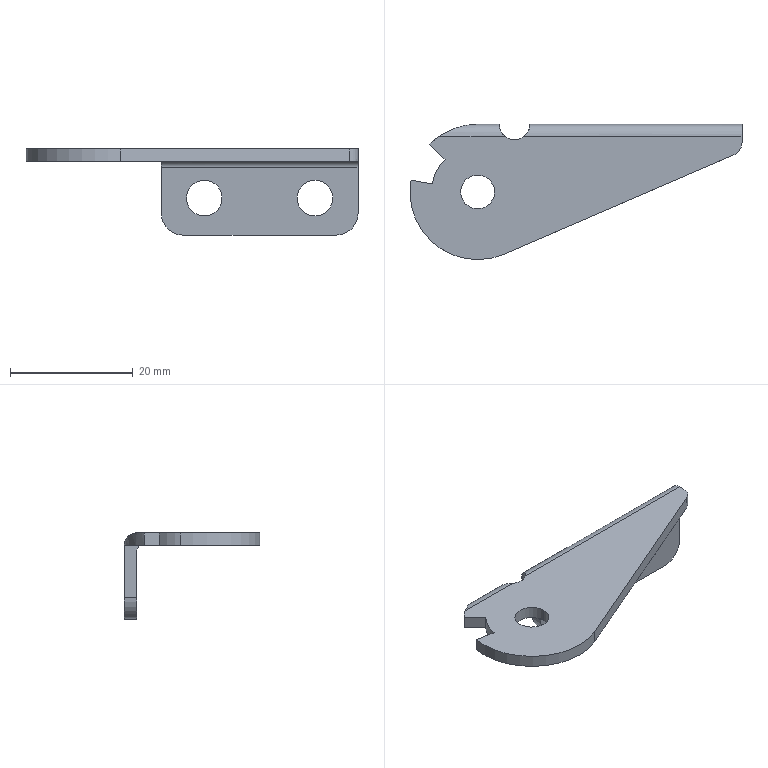Component | SolidWorks | MHPUS204-38-33-A-1_35-1 | 1 solid | 26 faces | box 54 x 22 x 14 mm | volume 2071 mm3 | cylinder 16 | plane 10 | commonest cylinder face diameters 5.8 x4 5.5 x2 4 x2 22 x2 7 x2 4.4 x1 15 x1 5 x1
STEP:
#1=COLOUR_RGB('',0.7922,0.8196,0.9333);
#2=FILL_AREA_STYLE_COLOUR('',#1);
#3=FILL_AREA_STYLE('',(#2));
#4=SURFACE_STYLE_FILL_AREA(#3);
#5=SURFACE_SIDE_STYLE('',(#4));
#6=SURFACE_STYLE_USAGE(.BOTH.,#5);
#7=PRESENTATION_STYLE_ASSIGNMENT((#6));
#8=CARTESIAN_POINT('',(20.594,-0.9055,3.138));
#9=VERTEX_POINT('',#8);
#10=CARTESIAN_POINT('',(20.81,-0.9055,3.138));
#11=VERTEX_POINT('',#10);
#12=CARTESIAN_POINT('',(20.702,-0.9055,3.138));
#13=DIRECTION('',(0.,0.,1.));
#14=DIRECTION('',(1.,0.,0.));
#15=AXIS2_PLACEMENT_3D('',#12,#13,#14);
#16=CIRCLE('',#15,0.1083);
#17=EDGE_CURVE('',#9,#11,#16,.T.);
#18=ORIENTED_EDGE('',*,*,#17,.F.);
#19=CARTESIAN_POINT('',(20.594,-0.9055,3.217));
#20=VERTEX_POINT('',#19);
#21=CARTESIAN_POINT('',(20.594,-0.9055,3.217));
#22=DIRECTION('',(0.,0.,1.));
#23=VECTOR('',#22,39.37);
#24=LINE('',#21,#23);
#25=EDGE_CURVE('',#9,#20,#24,.T.);
#26=ORIENTED_EDGE('',*,*,#25,.T.);
#27=CARTESIAN_POINT('',(20.81,-0.9055,3.217));
#28=VERTEX_POINT('',#27);
#29=CARTESIAN_POINT('',(20.702,-0.9055,3.217));
#30=DIRECTION('',(0.,0.,-1.));
#31=DIRECTION('',(1.,0.,0.));
#32=AXIS2_PLACEMENT_3D('',#29,#30,#31);
#33=CIRCLE('',#32,0.1083);
#34=EDGE_CURVE('',#28,#20,#33,.T.);
#35=ORIENTED_EDGE('',*,*,#34,.F.);
#36=CARTESIAN_POINT('',(20.81,-0.9055,3.217));
#37=DIRECTION('',(0.,0.,1.));
#38=VECTOR('',#37,39.37);
#39=LINE('',#36,#38);
#40=EDGE_CURVE('',#11,#28,#39,.T.);
#41=ORIENTED_EDGE('',*,*,#40,.F.);
#42=EDGE_LOOP('',(#18,#26,#35,#41));
#43=FACE_OUTER_BOUND('',#42,.T.);
#44=CARTESIAN_POINT('',(20.702,-0.9055,3.217));
#45=DIRECTION('',(0.,0.,1.));
#46=DIRECTION('',(1.,0.,0.));
#47=AXIS2_PLACEMENT_3D('',#44,#45,#46);
#48=CYLINDRICAL_SURFACE('',#47,0.1083);
#49=ADVANCED_FACE('',(#43),#48,.F.);
#50=CARTESIAN_POINT('',(21.411,-0.5512,2.787));
#51=VERTEX_POINT('',#50);
#52=CARTESIAN_POINT('',(21.411,-0.5512,3.016));
#53=VERTEX_POINT('',#52);
#54=CARTESIAN_POINT('',(21.411,-0.5512,2.902));
#55=DIRECTION('',(0.,1.,0.));
#56=DIRECTION('',(0.,0.,1.));
#57=AXIS2_PLACEMENT_3D('',#54,#55,#56);
#58=CIRCLE('',#57,0.1142);
#59=EDGE_CURVE('',#51,#53,#58,.T.);
#60=ORIENTED_EDGE('',*,*,#59,.F.);
#61=CARTESIAN_POINT('',(21.411,-0.4724,2.787));
#62=VERTEX_POINT('',#61);
#63=CARTESIAN_POINT('',(21.411,-0.3937,2.787));
#64=DIRECTION('',(0.,1.,0.));
#65=VECTOR('',#64,39.37);
#66=LINE('',#63,#65);
#67=EDGE_CURVE('',#51,#62,#66,.T.);
#68=ORIENTED_EDGE('',*,*,#67,.T.);
#69=CARTESIAN_POINT('',(21.411,-0.4724,3.016));
#70=VERTEX_POINT('',#69);
#71=CARTESIAN_POINT('',(21.411,-0.4724,2.902));
#72=DIRECTION('',(0.,-1.,0.));
#73=DIRECTION('',(0.,0.,1.));
#74=AXIS2_PLACEMENT_3D('',#71,#72,#73);
#75=CIRCLE('',#74,0.1142);
#76=EDGE_CURVE('',#70,#62,#75,.T.);
#77=ORIENTED_EDGE('',*,*,#76,.F.);
#78=CARTESIAN_POINT('',(21.411,-0.3937,3.016));
#79=DIRECTION('',(0.,1.,0.));
#80=VECTOR('',#79,39.37);
#81=LINE('',#78,#80);
#82=EDGE_CURVE('',#53,#70,#81,.T.);
#83=ORIENTED_EDGE('',*,*,#82,.F.);
#84=EDGE_LOOP('',(#60,#68,#77,#83));
#85=FACE_OUTER_BOUND('',#84,.T.);
#86=CARTESIAN_POINT('',(21.411,-0.3937,2.902));
#87=DIRECTION('',(0.,1.,0.));
#88=DIRECTION('',(0.,0.,1.));
#89=AXIS2_PLACEMENT_3D('',#86,#87,#88);
#90=CYLINDRICAL_SURFACE('',#89,0.1142);
#91=ADVANCED_FACE('',(#85),#90,.F.);
#92=CARTESIAN_POINT('',(22.119,-0.5512,2.787));
#93=VERTEX_POINT('',#92);
#94=CARTESIAN_POINT('',(22.119,-0.5512,3.016));
#95=VERTEX_POINT('',#94);
#96=CARTESIAN_POINT('',(22.119,-0.5512,2.902));
#97=DIRECTION('',(0.,1.,0.));
#98=DIRECTION('',(0.,0.,1.));
#99=AXIS2_PLACEMENT_3D('',#96,#97,#98);
#100=CIRCLE('',#99,0.1142);
#101=EDGE_CURVE('',#93,#95,#100,.T.);
#102=ORIENTED_EDGE('',*,*,#101,.F.);
#103=CARTESIAN_POINT('',(22.119,-0.4724,2.787));
#104=VERTEX_POINT('',#103);
#105=CARTESIAN_POINT('',(22.119,-0.3937,2.787));
#106=DIRECTION('',(0.,1.,0.));
#107=VECTOR('',#106,39.37);
#108=LINE('',#105,#107);
#109=EDGE_CURVE('',#93,#104,#108,.T.);
#110=ORIENTED_EDGE('',*,*,#109,.T.);
#111=CARTESIAN_POINT('',(22.119,-0.4724,3.016));
#112=VERTEX_POINT('',#111);
#113=CARTESIAN_POINT('',(22.119,-0.4724,2.902));
#114=DIRECTION('',(0.,-1.,0.));
#115=DIRECTION('',(0.,0.,1.));
#116=AXIS2_PLACEMENT_3D('',#113,#114,#115);
#117=CIRCLE('',#116,0.1142);
#118=EDGE_CURVE('',#112,#104,#117,.T.);
#119=ORIENTED_EDGE('',*,*,#118,.F.);
#120=CARTESIAN_POINT('',(22.119,-0.3937,3.016));
#121=DIRECTION('',(0.,1.,0.));
#122=VECTOR('',#121,39.37);
#123=LINE('',#120,#122);
#124=EDGE_CURVE('',#95,#112,#123,.T.);
#125=ORIENTED_EDGE('',*,*,#124,.F.);
#126=EDGE_LOOP('',(#102,#110,#119,#125));
#127=FACE_OUTER_BOUND('',#126,.T.);
#128=CARTESIAN_POINT('',(22.119,-0.3937,2.902));
#129=DIRECTION('',(0.,1.,0.));
#130=DIRECTION('',(0.,0.,1.));
#131=AXIS2_PLACEMENT_3D('',#128,#129,#130);
#132=CYLINDRICAL_SURFACE('',#131,0.1142);
#133=ADVANCED_FACE('',(#127),#132,.F.);
#134=CARTESIAN_POINT('',(22.395,-0.5512,3.217));
#135=VERTEX_POINT('',#134);
#136=CARTESIAN_POINT('',(22.395,-0.5887,3.217));
#137=VERTEX_POINT('',#136);
#138=CARTESIAN_POINT('',(22.395,-0.5887,3.217));
#139=DIRECTION('',(0.,-1.,0.));
#140=VECTOR('',#139,39.37);
#141=LINE('',#138,#140);
#142=EDGE_CURVE('',#135,#137,#141,.T.);
#143=ORIENTED_EDGE('',*,*,#142,.F.);
#144=CARTESIAN_POINT('',(20.997,-0.5512,3.217));
#145=VERTEX_POINT('',#144);
#146=CARTESIAN_POINT('',(20.702,-0.5512,3.217));
#147=DIRECTION('',(-1.,0.,0.));
#148=VECTOR('',#147,39.37);
#149=LINE('',#146,#148);
#150=EDGE_CURVE('',#135,#145,#149,.T.);
#151=ORIENTED_EDGE('',*,*,#150,.T.);
#152=CARTESIAN_POINT('',(20.879,-0.5512,3.217));
#153=VERTEX_POINT('',#152);
#154=CARTESIAN_POINT('',(20.938,-0.4724,3.217));
#155=DIRECTION('',(0.,0.,-1.));
#156=DIRECTION('',(1.,0.,0.));
#157=AXIS2_PLACEMENT_3D('',#154,#155,#156);
#158=CIRCLE('',#157,0.09843);
#159=EDGE_CURVE('',#145,#153,#158,.T.);
#160=ORIENTED_EDGE('',*,*,#159,.T.);
#161=CARTESIAN_POINT('',(20.453,-0.5512,3.217));
#162=VERTEX_POINT('',#161);
#163=CARTESIAN_POINT('',(20.702,-0.5512,3.217));
#164=DIRECTION('',(-1.,0.,0.));
#165=VECTOR('',#164,39.37);
#166=LINE('',#163,#165);
#167=EDGE_CURVE('',#153,#162,#166,.T.);
#168=ORIENTED_EDGE('',*,*,#167,.T.);
#169=CARTESIAN_POINT('',(20.396,-0.5993,3.217));
#170=VERTEX_POINT('',#169);
#171=CARTESIAN_POINT('',(20.702,-0.9055,3.217));
#172=DIRECTION('',(0.,0.,1.));
#173=DIRECTION('',(1.,0.,0.));
#174=AXIS2_PLACEMENT_3D('',#171,#172,#173);
#175=CIRCLE('',#174,0.4331);
#176=EDGE_CURVE('',#162,#170,#175,.T.);
#177=ORIENTED_EDGE('',*,*,#176,.T.);
#178=CARTESIAN_POINT('',(20.493,-0.6967,3.217));
#179=VERTEX_POINT('',#178);
#180=CARTESIAN_POINT('',(20.396,-0.5993,3.217));
#181=DIRECTION('',(0.7071,-0.7071,0.));
#182=VECTOR('',#181,39.37);
#183=LINE('',#180,#182);
#184=EDGE_CURVE('',#170,#179,#183,.T.);
#185=ORIENTED_EDGE('',*,*,#184,.T.);
#186=CARTESIAN_POINT('',(20.411,-0.8542,3.217));
#187=VERTEX_POINT('',#186);
#188=CARTESIAN_POINT('',(20.702,-0.9055,3.217));
#189=DIRECTION('',(0.,0.,1.));
#190=DIRECTION('',(1.,0.,0.));
#191=AXIS2_PLACEMENT_3D('',#188,#189,#190);
#192=CIRCLE('',#191,0.2953);
#193=EDGE_CURVE('',#179,#187,#192,.T.);
#194=ORIENTED_EDGE('',*,*,#193,.T.);
#195=CARTESIAN_POINT('',(20.276,-0.8303,3.217));
#196=VERTEX_POINT('',#195);
#197=CARTESIAN_POINT('',(20.411,-0.8542,3.217));
#198=DIRECTION('',(-0.9848,0.1736,0.));
#199=VECTOR('',#198,39.37);
#200=LINE('',#197,#199);
#201=EDGE_CURVE('',#187,#196,#200,.T.);
#202=ORIENTED_EDGE('',*,*,#201,.T.);
#203=CARTESIAN_POINT('',(20.874,-1.303,3.217));
#204=VERTEX_POINT('',#203);
#205=CARTESIAN_POINT('',(20.702,-0.9055,3.217));
#206=DIRECTION('',(0.,0.,1.));
#207=DIRECTION('',(1.,0.,0.));
#208=AXIS2_PLACEMENT_3D('',#205,#206,#207);
#209=CIRCLE('',#208,0.4331);
#210=EDGE_CURVE('',#196,#204,#209,.T.);
#211=ORIENTED_EDGE('',*,*,#210,.T.);
#212=CARTESIAN_POINT('',(22.343,-0.6683,3.217));
#213=VERTEX_POINT('',#212);
#214=CARTESIAN_POINT('',(20.874,-1.303,3.217));
#215=DIRECTION('',(0.9179,0.3967,0.));
#216=VECTOR('',#215,39.37);
#217=LINE('',#214,#216);
#218=EDGE_CURVE('',#204,#213,#217,.T.);
#219=ORIENTED_EDGE('',*,*,#218,.T.);
#220=CARTESIAN_POINT('',(22.308,-0.5887,3.217));
#221=DIRECTION('',(0.,0.,1.));
#222=DIRECTION('',(1.,0.,0.));
#223=AXIS2_PLACEMENT_3D('',#220,#221,#222);
#224=CIRCLE('',#223,0.08661);
#225=EDGE_CURVE('',#213,#137,#224,.T.);
#226=ORIENTED_EDGE('',*,*,#225,.T.);
#227=EDGE_LOOP('',(#143,#151,#160,#168,#177,#185,#194,#202,#211,#219,#226));
#228=FACE_OUTER_BOUND('',#227,.T.);
#229=ORIENTED_EDGE('',*,*,#34,.T.);
#230=CARTESIAN_POINT('',(20.702,-0.9055,3.217));
#231=DIRECTION('',(0.,0.,-1.));
#232=DIRECTION('',(1.,0.,0.));
#233=AXIS2_PLACEMENT_3D('',#230,#231,#232);
#234=CIRCLE('',#233,0.1083);
#235=EDGE_CURVE('',#20,#28,#234,.T.);
#236=ORIENTED_EDGE('',*,*,#235,.T.);
#237=EDGE_LOOP('',(#229,#236));
#238=FACE_BOUND('',#237,.T.);
#239=CARTESIAN_POINT('',(20.702,-1.339,3.217));
#240=DIRECTION('',(0.,0.,1.));
#241=DIRECTION('',(1.,0.,0.));
#242=AXIS2_PLACEMENT_3D('',#239,#240,#241);
#243=PLANE('',#242);
#244=ADVANCED_FACE('',(#228,#238),#243,.T.);
#245=CARTESIAN_POINT('',(22.395,-0.4724,3.138));
#246=VERTEX_POINT('',#245);
#247=CARTESIAN_POINT('',(21.135,-0.4724,3.138));
#248=VERTEX_POINT('',#247);
#249=CARTESIAN_POINT('',(23.261,-0.4724,3.138));
#250=DIRECTION('',(-1.,0.,0.));
#251=VECTOR('',#250,39.37);
#252=LINE('',#249,#251);
#253=EDGE_CURVE('',#246,#248,#252,.T.);
#254=ORIENTED_EDGE('',*,*,#253,.T.);
#255=CARTESIAN_POINT('',(21.037,-0.4724,3.138));
#256=VERTEX_POINT('',#255);
#257=CARTESIAN_POINT('',(23.261,-0.4724,3.138));
#258=DIRECTION('',(-1.,0.,0.));
#259=VECTOR('',#258,39.37);
#260=LINE('',#257,#259);
#261=EDGE_CURVE('',#248,#256,#260,.T.);
#262=ORIENTED_EDGE('',*,*,#261,.T.);
#263=CARTESIAN_POINT('',(21.037,-0.4724,3.138));
#264=CARTESIAN_POINT('',(21.037,-0.4724,3.143));
#265=CARTESIAN_POINT('',(21.037,-0.4731,3.149));
#266=CARTESIAN_POINT('',(21.037,-0.4755,3.16));
#267=CARTESIAN_POINT('',(21.037,-0.4773,3.166));
#268=CARTESIAN_POINT('',(21.036,-0.482,3.176));
#269=CARTESIAN_POINT('',(21.036,-0.4849,3.181));
#270=CARTESIAN_POINT('',(21.035,-0.4917,3.19));
#271=CARTESIAN_POINT('',(21.034,-0.4955,3.194));
#272=CARTESIAN_POINT('',(21.032,-0.5038,3.201));
#273=CARTESIAN_POINT('',(21.03,-0.5084,3.204));
#274=CARTESIAN_POINT('',(21.026,-0.5175,3.209));
#275=CARTESIAN_POINT('',(21.023,-0.5222,3.211));
#276=CARTESIAN_POINT('',(21.014,-0.5359,3.216));
#277=CARTESIAN_POINT('',(21.006,-0.5443,3.217));
#278=CARTESIAN_POINT('',(20.997,-0.5512,3.217));
#279=B_SPLINE_CURVE_WITH_KNOTS('',3,(#263,#264,#265,#266,#267,#268,#269,#270,#271,#272,#273,#274,#275,#276,#277,#278),.UNSPECIFIED.,.F.,.F.,(4,2,2,2,2,2,2,4),(0.,0.0004284,0.0008569,0.001285,0.001714,0.002142,0.002571,0.003428),.UNSPECIFIED.);
#280=EDGE_CURVE('',#256,#145,#279,.T.);
#281=ORIENTED_EDGE('',*,*,#280,.T.);
#282=ORIENTED_EDGE('',*,*,#150,.F.);
#283=CARTESIAN_POINT('',(22.395,-0.5512,3.138));
#284=DIRECTION('',(-1.,0.,0.));
#285=DIRECTION('',(0.,0.,-1.));
#286=AXIS2_PLACEMENT_3D('',#283,#284,#285);
#287=CIRCLE('',#286,0.07874);
#288=EDGE_CURVE('',#135,#246,#287,.T.);
#289=ORIENTED_EDGE('',*,*,#288,.T.);
#290=EDGE_LOOP('',(#254,#262,#281,#282,#289));
#291=FACE_OUTER_BOUND('',#290,.T.);
#292=CARTESIAN_POINT('',(23.261,-0.5512,3.138));
#293=DIRECTION('',(1.,0.,0.));
#294=DIRECTION('',(0.,0.,-1.));
#295=AXIS2_PLACEMENT_3D('',#292,#293,#294);
#296=CYLINDRICAL_SURFACE('',#295,0.07874);
#297=ADVANCED_FACE('',(#291),#296,.T.);
#298=CARTESIAN_POINT('',(22.343,-0.6683,3.138));
#299=VERTEX_POINT('',#298);
#300=CARTESIAN_POINT('',(22.343,-0.6683,3.217));
#301=DIRECTION('',(0.,0.,-1.));
#302=VECTOR('',#301,39.37);
#303=LINE('',#300,#302);
#304=EDGE_CURVE('',#213,#299,#303,.T.);
#305=ORIENTED_EDGE('',*,*,#304,.T.);
#306=CARTESIAN_POINT('',(22.395,-0.5906,3.138));
#307=VERTEX_POINT('',#306);
#308=CARTESIAN_POINT('',(22.308,-0.5887,3.138));
#309=DIRECTION('',(0.,0.,1.));
#310=DIRECTION('',(1.,0.,0.));
#311=AXIS2_PLACEMENT_3D('',#308,#309,#310);
#312=CIRCLE('',#311,0.08661);
#313=EDGE_CURVE('',#299,#307,#312,.T.);
#314=ORIENTED_EDGE('',*,*,#313,.T.);
#315=CARTESIAN_POINT('',(22.395,-0.5887,3.138));
#316=VERTEX_POINT('',#315);
#317=CARTESIAN_POINT('',(22.395,-0.5906,3.138));
#318=CARTESIAN_POINT('',(22.395,-0.5899,3.138));
#319=CARTESIAN_POINT('',(22.395,-0.5893,3.138));
#320=CARTESIAN_POINT('',(22.395,-0.5887,3.138));
#321=B_SPLINE_CURVE_WITH_KNOTS('',3,(#317,#318,#319,#320),.UNSPECIFIED.,.F.,.F.,(4,4),(0.,0.0000459),.UNSPECIFIED.);
#322=EDGE_CURVE('',#307,#316,#321,.T.);
#323=ORIENTED_EDGE('',*,*,#322,.T.);
#324=CARTESIAN_POINT('',(22.395,-0.5887,3.217));
#325=DIRECTION('',(0.,0.,1.));
#326=VECTOR('',#325,39.37);
#327=LINE('',#324,#326);
#328=EDGE_CURVE('',#316,#137,#327,.T.);
#329=ORIENTED_EDGE('',*,*,#328,.T.);
#330=ORIENTED_EDGE('',*,*,#225,.F.);
#331=EDGE_LOOP('',(#305,#314,#323,#329,#330));
#332=FACE_OUTER_BOUND('',#331,.T.);
#333=CARTESIAN_POINT('',(22.308,-0.5887,3.217));
#334=DIRECTION('',(0.,0.,1.));
#335=DIRECTION('',(1.,0.,0.));
#336=AXIS2_PLACEMENT_3D('',#333,#334,#335);
#337=CYLINDRICAL_SURFACE('',#336,0.08661);
#338=ADVANCED_FACE('',(#332),#337,.T.);
#339=ORIENTED_EDGE('',*,*,#218,.F.);
#340=CARTESIAN_POINT('',(20.874,-1.303,3.138));
#341=VERTEX_POINT('',#340);
#342=CARTESIAN_POINT('',(20.874,-1.303,3.217));
#343=DIRECTION('',(0.,0.,-1.));
#344=VECTOR('',#343,39.37);
#345=LINE('',#342,#344);
#346=EDGE_CURVE('',#204,#341,#345,.T.);
#347=ORIENTED_EDGE('',*,*,#346,.T.);
#348=CARTESIAN_POINT('',(20.874,-1.303,3.138));
#349=DIRECTION('',(0.9179,0.3967,0.));
#350=VECTOR('',#349,39.37);
#351=LINE('',#348,#350);
#352=EDGE_CURVE('',#341,#299,#351,.T.);
#353=ORIENTED_EDGE('',*,*,#352,.T.);
#354=ORIENTED_EDGE('',*,*,#304,.F.);
#355=EDGE_LOOP('',(#339,#347,#353,#354));
#356=FACE_OUTER_BOUND('',#355,.T.);
#357=CARTESIAN_POINT('',(20.874,-1.303,3.217));
#358=DIRECTION('',(0.3967,-0.9179,0.));
#359=DIRECTION('',(0.9179,0.3967,0.));
#360=AXIS2_PLACEMENT_3D('',#357,#358,#359);
#361=PLANE('',#360);
#362=ADVANCED_FACE('',(#356),#361,.T.);
#363=ORIENTED_EDGE('',*,*,#210,.F.);
#364=CARTESIAN_POINT('',(20.276,-0.8303,3.138));
#365=VERTEX_POINT('',#364);
#366=CARTESIAN_POINT('',(20.276,-0.8303,3.217));
#367=DIRECTION('',(0.,0.,-1.));
#368=VECTOR('',#367,39.37);
#369=LINE('',#366,#368);
#370=EDGE_CURVE('',#196,#365,#369,.T.);
#371=ORIENTED_EDGE('',*,*,#370,.T.);
#372=CARTESIAN_POINT('',(20.702,-0.9055,3.138));
#373=DIRECTION('',(0.,0.,1.));
#374=DIRECTION('',(1.,0.,0.));
#375=AXIS2_PLACEMENT_3D('',#372,#373,#374);
#376=CIRCLE('',#375,0.4331);
#377=EDGE_CURVE('',#365,#341,#376,.T.);
#378=ORIENTED_EDGE('',*,*,#377,.T.);
#379=ORIENTED_EDGE('',*,*,#346,.F.);
#380=EDGE_LOOP('',(#363,#371,#378,#379));
#381=FACE_OUTER_BOUND('',#380,.T.);
#382=CARTESIAN_POINT('',(20.702,-0.9055,3.217));
#383=DIRECTION('',(0.,0.,1.));
#384=DIRECTION('',(1.,0.,0.));
#385=AXIS2_PLACEMENT_3D('',#382,#383,#384);
#386=CYLINDRICAL_SURFACE('',#385,0.4331);
#387=ADVANCED_FACE('',(#381),#386,.T.);
#388=ORIENTED_EDGE('',*,*,#201,.F.);
#389=CARTESIAN_POINT('',(20.411,-0.8542,3.138));
#390=VERTEX_POINT('',#389);
#391=CARTESIAN_POINT('',(20.411,-0.8542,3.217));
#392=DIRECTION('',(0.,0.,-1.));
#393=VECTOR('',#392,39.37);
#394=LINE('',#391,#393);
#395=EDGE_CURVE('',#187,#390,#394,.T.);
#396=ORIENTED_EDGE('',*,*,#395,.T.);
#397=CARTESIAN_POINT('',(20.411,-0.8542,3.138));
#398=DIRECTION('',(-0.9848,0.1736,0.));
#399=VECTOR('',#398,39.37);
#400=LINE('',#397,#399);
#401=EDGE_CURVE('',#390,#365,#400,.T.);
#402=ORIENTED_EDGE('',*,*,#401,.T.);
#403=ORIENTED_EDGE('',*,*,#370,.F.);
#404=EDGE_LOOP('',(#388,#396,#402,#403));
#405=FACE_OUTER_BOUND('',#404,.T.);
#406=CARTESIAN_POINT('',(20.411,-0.8542,3.217));
#407=DIRECTION('',(0.1736,0.9848,0.));
#408=DIRECTION('',(-0.9848,0.1736,0.));
#409=AXIS2_PLACEMENT_3D('',#406,#407,#408);
#410=PLANE('',#409);
#411=ADVANCED_FACE('',(#405),#410,.T.);
#412=ORIENTED_EDGE('',*,*,#193,.F.);
#413=CARTESIAN_POINT('',(20.493,-0.6967,3.138));
#414=VERTEX_POINT('',#413);
#415=CARTESIAN_POINT('',(20.493,-0.6967,3.217));
#416=DIRECTION('',(0.,0.,-1.));
#417=VECTOR('',#416,39.37);
#418=LINE('',#415,#417);
#419=EDGE_CURVE('',#179,#414,#418,.T.);
#420=ORIENTED_EDGE('',*,*,#419,.T.);
#421=CARTESIAN_POINT('',(20.702,-0.9055,3.138));
#422=DIRECTION('',(0.,0.,1.));
#423=DIRECTION('',(1.,0.,0.));
#424=AXIS2_PLACEMENT_3D('',#421,#422,#423);
#425=CIRCLE('',#424,0.2953);
#426=EDGE_CURVE('',#414,#390,#425,.T.);
#427=ORIENTED_EDGE('',*,*,#426,.T.);
#428=ORIENTED_EDGE('',*,*,#395,.F.);
#429=EDGE_LOOP('',(#412,#420,#427,#428));
#430=FACE_OUTER_BOUND('',#429,.T.);
#431=CARTESIAN_POINT('',(20.702,-0.9055,3.217));
#432=DIRECTION('',(0.,0.,1.));
#433=DIRECTION('',(1.,0.,0.));
#434=AXIS2_PLACEMENT_3D('',#431,#432,#433);
#435=CYLINDRICAL_SURFACE('',#434,0.2953);
#436=ADVANCED_FACE('',(#430),#435,.T.);
#437=ORIENTED_EDGE('',*,*,#184,.F.);
#438=CARTESIAN_POINT('',(20.396,-0.5993,3.138));
#439=VERTEX_POINT('',#438);
#440=CARTESIAN_POINT('',(20.396,-0.5993,3.217));
#441=DIRECTION('',(0.,0.,-1.));
#442=VECTOR('',#441,39.37);
#443=LINE('',#440,#442);
#444=EDGE_CURVE('',#170,#439,#443,.T.);
#445=ORIENTED_EDGE('',*,*,#444,.T.);
#446=CARTESIAN_POINT('',(20.396,-0.5993,3.138));
#447=DIRECTION('',(0.7071,-0.7071,0.));
#448=VECTOR('',#447,39.37);
#449=LINE('',#446,#448);
#450=EDGE_CURVE('',#439,#414,#449,.T.);
#451=ORIENTED_EDGE('',*,*,#450,.T.);
#452=ORIENTED_EDGE('',*,*,#419,.F.);
#453=EDGE_LOOP('',(#437,#445,#451,#452));
#454=FACE_OUTER_BOUND('',#453,.T.);
#455=CARTESIAN_POINT('',(20.396,-0.5993,3.217));
#456=DIRECTION('',(-0.7071,-0.7071,0.));
#457=DIRECTION('',(0.7071,-0.7071,0.));
#458=AXIS2_PLACEMENT_3D('',#455,#456,#457);
#459=PLANE('',#458);
#460=ADVANCED_FACE('',(#454),#459,.T.);
#461=ORIENTED_EDGE('',*,*,#176,.F.);
#462=CARTESIAN_POINT('',(20.702,-0.4724,3.138));
#463=VERTEX_POINT('',#462);
#464=CARTESIAN_POINT('',(20.453,-0.5512,3.217));
#465=CARTESIAN_POINT('',(20.472,-0.5377,3.217));
#466=CARTESIAN_POINT('',(20.492,-0.5261,3.213));
#467=CARTESIAN_POINT('',(20.523,-0.5111,3.206));
#468=CARTESIAN_POINT('',(20.533,-0.5066,3.203));
#469=CARTESIAN_POINT('',(20.554,-0.4984,3.196));
#470=CARTESIAN_POINT('',(20.564,-0.4948,3.193));
#471=CARTESIAN_POINT('',(20.596,-0.4852,3.182));
#472=CARTESIAN_POINT('',(20.617,-0.4804,3.174));
#473=CARTESIAN_POINT('',(20.649,-0.4756,3.16));
#474=CARTESIAN_POINT('',(20.659,-0.4744,3.156));
#475=CARTESIAN_POINT('',(20.681,-0.4728,3.147));
#476=CARTESIAN_POINT('',(20.691,-0.4724,3.142));
#477=CARTESIAN_POINT('',(20.702,-0.4724,3.138));
#478=B_SPLINE_CURVE_WITH_KNOTS('',3,(#464,#465,#466,#467,#468,#469,#470,#471,#472,#473,#474,#475,#476,#477),.UNSPECIFIED.,.F.,.F.,(4,2,2,2,2,2,4),(0.,0.001765,0.002648,0.003531,0.005296,0.006179,0.007061),.UNSPECIFIED.);
#479=EDGE_CURVE('',#162,#463,#478,.T.);
#480=ORIENTED_EDGE('',*,*,#479,.T.);
#481=CARTESIAN_POINT('',(20.702,-0.9055,3.138));
#482=DIRECTION('',(0.,0.,1.));
#483=DIRECTION('',(1.,0.,0.));
#484=AXIS2_PLACEMENT_3D('',#481,#482,#483);
#485=CIRCLE('',#484,0.4331);
#486=EDGE_CURVE('',#463,#439,#485,.T.);
#487=ORIENTED_EDGE('',*,*,#486,.T.);
#488=ORIENTED_EDGE('',*,*,#444,.F.);
#489=EDGE_LOOP('',(#461,#480,#487,#488));
#490=FACE_OUTER_BOUND('',#489,.T.);
#491=CARTESIAN_POINT('',(20.702,-0.9055,3.217));
#492=DIRECTION('',(0.,0.,1.));
#493=DIRECTION('',(1.,0.,0.));
#494=AXIS2_PLACEMENT_3D('',#491,#492,#493);
#495=CYLINDRICAL_SURFACE('',#494,0.4331);
#496=ADVANCED_FACE('',(#490),#495,.T.);
#497=ORIENTED_EDGE('',*,*,#479,.F.);
#498=ORIENTED_EDGE('',*,*,#167,.F.);
#499=CARTESIAN_POINT('',(20.84,-0.4724,3.138));
#500=VERTEX_POINT('',#499);
#501=CARTESIAN_POINT('',(20.879,-0.5512,3.217));
#502=CARTESIAN_POINT('',(20.875,-0.5478,3.217));
#503=CARTESIAN_POINT('',(20.871,-0.544,3.216));
#504=CARTESIAN_POINT('',(20.863,-0.5359,3.215));
#505=CARTESIAN_POINT('',(20.859,-0.5314,3.214));
#506=CARTESIAN_POINT('',(20.853,-0.5224,3.211));
#507=CARTESIAN_POINT('',(20.851,-0.5177,3.209));
#508=CARTESIAN_POINT('',(20.847,-0.5085,3.204));
#509=CARTESIAN_POINT('',(20.845,-0.504,3.201));
#510=CARTESIAN_POINT('',(20.843,-0.4957,3.194));
#511=CARTESIAN_POINT('',(20.842,-0.4917,3.19));
#512=CARTESIAN_POINT('',(20.841,-0.485,3.181));
#513=CARTESIAN_POINT('',(20.84,-0.482,3.176));
#514=CARTESIAN_POINT('',(20.84,-0.4773,3.166));
#515=CARTESIAN_POINT('',(20.84,-0.4755,3.16));
#516=CARTESIAN_POINT('',(20.84,-0.4731,3.149));
#517=CARTESIAN_POINT('',(20.84,-0.4724,3.143));
#518=CARTESIAN_POINT('',(20.84,-0.4724,3.138));
#519=B_SPLINE_CURVE_WITH_KNOTS('',3,(#501,#502,#503,#504,#505,#506,#507,#508,#509,#510,#511,#512,#513,#514,#515,#516,#517,#518),.UNSPECIFIED.,.F.,.F.,(4,2,2,2,2,2,2,2,4),(0.,0.0004287,0.0008574,0.001286,0.001715,0.002144,0.002572,0.003001,0.00343),.UNSPECIFIED.);
#520=EDGE_CURVE('',#153,#500,#519,.T.);
#521=ORIENTED_EDGE('',*,*,#520,.T.);
#522=CARTESIAN_POINT('',(23.261,-0.4724,3.138));
#523=DIRECTION('',(-1.,0.,0.));
#524=VECTOR('',#523,39.37);
#525=LINE('',#522,#524);
#526=EDGE_CURVE('',#500,#463,#525,.T.);
#527=ORIENTED_EDGE('',*,*,#526,.T.);
#528=EDGE_LOOP('',(#497,#498,#521,#527));
#529=FACE_OUTER_BOUND('',#528,.T.);
#530=CARTESIAN_POINT('',(23.261,-0.5512,3.138));
#531=DIRECTION('',(1.,0.,0.));
#532=DIRECTION('',(0.,0.,-1.));
#533=AXIS2_PLACEMENT_3D('',#530,#531,#532);
#534=CYLINDRICAL_SURFACE('',#533,0.07874);
#535=ADVANCED_FACE('',(#529),#534,.T.);
#536=CARTESIAN_POINT('',(20.938,-0.4724,3.138));
#537=DIRECTION('',(0.,0.,1.));
#538=DIRECTION('',(1.,0.,0.));
#539=AXIS2_PLACEMENT_3D('',#536,#537,#538);
#540=CIRCLE('',#539,0.09843);
#541=EDGE_CURVE('',#500,#256,#540,.T.);
#542=ORIENTED_EDGE('',*,*,#541,.F.);
#543=ORIENTED_EDGE('',*,*,#520,.F.);
#544=ORIENTED_EDGE('',*,*,#159,.F.);
#545=ORIENTED_EDGE('',*,*,#280,.F.);
#546=EDGE_LOOP('',(#542,#543,#544,#545));
#547=FACE_OUTER_BOUND('',#546,.T.);
#548=CARTESIAN_POINT('',(20.938,-0.4724,3.217));
#549=DIRECTION('',(0.,0.,1.));
#550=DIRECTION('',(1.,0.,0.));
#551=AXIS2_PLACEMENT_3D('',#548,#549,#550);
#552=CYLINDRICAL_SURFACE('',#551,0.09843);
#553=ADVANCED_FACE('',(#547),#552,.F.);
#554=ORIENTED_EDGE('',*,*,#25,.F.);
#555=CARTESIAN_POINT('',(20.702,-0.9055,3.138));
#556=DIRECTION('',(0.,0.,1.));
#557=DIRECTION('',(1.,0.,0.));
#558=AXIS2_PLACEMENT_3D('',#555,#556,#557);
#559=CIRCLE('',#558,0.1083);
#560=EDGE_CURVE('',#11,#9,#559,.T.);
#561=ORIENTED_EDGE('',*,*,#560,.F.);
#562=ORIENTED_EDGE('',*,*,#40,.T.);
#563=ORIENTED_EDGE('',*,*,#235,.F.);
#564=EDGE_LOOP('',(#554,#561,#562,#563));
#565=FACE_OUTER_BOUND('',#564,.T.);
#566=CARTESIAN_POINT('',(20.702,-0.9055,3.217));
#567=DIRECTION('',(0.,0.,1.));
#568=DIRECTION('',(1.,0.,0.));
#569=AXIS2_PLACEMENT_3D('',#566,#567,#568);
#570=CYLINDRICAL_SURFACE('',#569,0.1083);
#571=ADVANCED_FACE('',(#565),#570,.F.);
#572=ORIENTED_EDGE('',*,*,#560,.T.);
#573=ORIENTED_EDGE('',*,*,#17,.T.);
#574=EDGE_LOOP('',(#572,#573));
#575=FACE_BOUND('',#574,.T.);
#576=ORIENTED_EDGE('',*,*,#261,.F.);
#577=CARTESIAN_POINT('',(21.135,-0.5906,3.138));
#578=VERTEX_POINT('',#577);
#579=CARTESIAN_POINT('',(21.135,-0.5906,3.138));
#580=DIRECTION('',(0.,1.,0.));
#581=VECTOR('',#580,39.37);
#582=LINE('',#579,#581);
#583=EDGE_CURVE('',#578,#248,#582,.T.);
#584=ORIENTED_EDGE('',*,*,#583,.F.);
#585=CARTESIAN_POINT('',(23.261,-0.5906,3.138));
#586=DIRECTION('',(-1.,0.,0.));
#587=VECTOR('',#586,39.37);
#588=LINE('',#585,#587);
#589=EDGE_CURVE('',#307,#578,#588,.T.);
#590=ORIENTED_EDGE('',*,*,#589,.F.);
#591=ORIENTED_EDGE('',*,*,#313,.F.);
#592=ORIENTED_EDGE('',*,*,#352,.F.);
#593=ORIENTED_EDGE('',*,*,#377,.F.);
#594=ORIENTED_EDGE('',*,*,#401,.F.);
#595=ORIENTED_EDGE('',*,*,#426,.F.);
#596=ORIENTED_EDGE('',*,*,#450,.F.);
#597=ORIENTED_EDGE('',*,*,#486,.F.);
#598=ORIENTED_EDGE('',*,*,#526,.F.);
#599=ORIENTED_EDGE('',*,*,#541,.T.);
#600=EDGE_LOOP('',(#576,#584,#590,#591,#592,#593,#594,#595,#596,#597,#598,#599));
#601=FACE_OUTER_BOUND('',#600,.T.);
#602=CARTESIAN_POINT('',(23.261,-0.5906,3.138));
#603=DIRECTION('',(0.,0.,1.));
#604=DIRECTION('',(1.,0.,0.));
#605=AXIS2_PLACEMENT_3D('',#602,#603,#604);
#606=PLANE('',#605);
#607=ADVANCED_FACE('',(#575,#601),#606,.F.);
#608=ORIENTED_EDGE('',*,*,#253,.F.);
#609=CARTESIAN_POINT('',(22.395,-0.4724,2.803));
#610=VERTEX_POINT('',#609);
#611=CARTESIAN_POINT('',(22.395,-0.4724,3.217));
#612=DIRECTION('',(0.,0.,-1.));
#613=VECTOR('',#612,39.37);
#614=LINE('',#611,#613);
#615=EDGE_CURVE('',#246,#610,#614,.T.);
#616=ORIENTED_EDGE('',*,*,#615,.T.);
#617=CARTESIAN_POINT('',(22.257,-0.4724,2.665));
#618=VERTEX_POINT('',#617);
#619=CARTESIAN_POINT('',(22.257,-0.4724,2.803));
#620=DIRECTION('',(0.,1.,0.));
#621=DIRECTION('',(0.,0.,-1.));
#622=AXIS2_PLACEMENT_3D('',#619,#620,#621);
#623=CIRCLE('',#622,0.1378);
#624=EDGE_CURVE('',#610,#618,#623,.T.);
#625=ORIENTED_EDGE('',*,*,#624,.T.);
#626=CARTESIAN_POINT('',(21.273,-0.4724,2.665));
#627=VERTEX_POINT('',#626);
#628=CARTESIAN_POINT('',(22.395,-0.4724,2.665));
#629=DIRECTION('',(-1.,0.,0.));
#630=VECTOR('',#629,39.37);
#631=LINE('',#628,#630);
#632=EDGE_CURVE('',#618,#627,#631,.T.);
#633=ORIENTED_EDGE('',*,*,#632,.T.);
#634=CARTESIAN_POINT('',(21.135,-0.4724,2.803));
#635=VERTEX_POINT('',#634);
#636=CARTESIAN_POINT('',(21.273,-0.4724,2.803));
#637=DIRECTION('',(0.,1.,0.));
#638=DIRECTION('',(0.,0.,-1.));
#639=AXIS2_PLACEMENT_3D('',#636,#637,#638);
#640=CIRCLE('',#639,0.1378);
#641=EDGE_CURVE('',#627,#635,#640,.T.);
#642=ORIENTED_EDGE('',*,*,#641,.T.);
#643=CARTESIAN_POINT('',(21.135,-0.4724,3.217));
#644=DIRECTION('',(0.,0.,1.));
#645=VECTOR('',#644,39.37);
#646=LINE('',#643,#645);
#647=EDGE_CURVE('',#635,#248,#646,.T.);
#648=ORIENTED_EDGE('',*,*,#647,.T.);
#649=EDGE_LOOP('',(#608,#616,#625,#633,#642,#648));
#650=FACE_OUTER_BOUND('',#649,.T.);
#651=ORIENTED_EDGE('',*,*,#76,.T.);
#652=CARTESIAN_POINT('',(21.411,-0.4724,2.902));
#653=DIRECTION('',(0.,-1.,0.));
#654=DIRECTION('',(0.,0.,1.));
#655=AXIS2_PLACEMENT_3D('',#652,#653,#654);
#656=CIRCLE('',#655,0.1142);
#657=EDGE_CURVE('',#62,#70,#656,.T.);
#658=ORIENTED_EDGE('',*,*,#657,.T.);
#659=EDGE_LOOP('',(#651,#658));
#660=FACE_BOUND('',#659,.T.);
#661=ORIENTED_EDGE('',*,*,#118,.T.);
#662=CARTESIAN_POINT('',(22.119,-0.4724,2.902));
#663=DIRECTION('',(0.,-1.,0.));
#664=DIRECTION('',(0.,0.,1.));
#665=AXIS2_PLACEMENT_3D('',#662,#663,#664);
#666=CIRCLE('',#665,0.1142);
#667=EDGE_CURVE('',#104,#112,#666,.T.);
#668=ORIENTED_EDGE('',*,*,#667,.T.);
#669=EDGE_LOOP('',(#661,#668));
#670=FACE_BOUND('',#669,.T.);
#671=CARTESIAN_POINT('',(22.395,-0.4724,3.217));
#672=DIRECTION('',(0.,1.,0.));
#673=DIRECTION('',(0.,0.,1.));
#674=AXIS2_PLACEMENT_3D('',#671,#672,#673);
#675=PLANE('',#674);
#676=ADVANCED_FACE('',(#650,#660,#670),#675,.T.);
#677=CARTESIAN_POINT('',(22.395,-0.5512,3.098));
#678=VERTEX_POINT('',#677);
#679=CARTESIAN_POINT('',(22.395,-0.5906,3.098));
#680=DIRECTION('',(-1.,0.,0.));
#681=DIRECTION('',(0.,-0.,-1.));
#682=AXIS2_PLACEMENT_3D('',#679,#680,#681);
#683=CIRCLE('',#682,0.03937);
#684=EDGE_CURVE('',#316,#678,#683,.T.);
#685=ORIENTED_EDGE('',*,*,#684,.T.);
#686=CARTESIAN_POINT('',(22.395,-0.5512,2.803));
#687=VERTEX_POINT('',#686);
#688=CARTESIAN_POINT('',(22.395,-0.5512,3.217));
#689=DIRECTION('',(0.,0.,-1.));
#690=VECTOR('',#689,39.37);
#691=LINE('',#688,#690);
#692=EDGE_CURVE('',#678,#687,#691,.T.);
#693=ORIENTED_EDGE('',*,*,#692,.T.);
#694=CARTESIAN_POINT('',(22.395,-0.5887,2.803));
#695=DIRECTION('',(0.,1.,0.));
#696=VECTOR('',#695,39.37);
#697=LINE('',#694,#696);
#698=EDGE_CURVE('',#687,#610,#697,.T.);
#699=ORIENTED_EDGE('',*,*,#698,.T.);
#700=ORIENTED_EDGE('',*,*,#615,.F.);
#701=ORIENTED_EDGE('',*,*,#288,.F.);
#702=ORIENTED_EDGE('',*,*,#142,.T.);
#703=ORIENTED_EDGE('',*,*,#328,.F.);
#704=EDGE_LOOP('',(#685,#693,#699,#700,#701,#702,#703));
#705=FACE_OUTER_BOUND('',#704,.T.);
#706=CARTESIAN_POINT('',(22.395,-0.5887,3.217));
#707=DIRECTION('',(1.,0.,0.));
#708=DIRECTION('',(0.,0.,-1.));
#709=AXIS2_PLACEMENT_3D('',#706,#707,#708);
#710=PLANE('',#709);
#711=ADVANCED_FACE('',(#705),#710,.T.);
#712=CARTESIAN_POINT('',(21.135,-0.5512,3.098));
#713=VERTEX_POINT('',#712);
#714=CARTESIAN_POINT('',(21.135,-0.5906,3.098));
#715=DIRECTION('',(-1.,0.,0.));
#716=DIRECTION('',(0.,0.,-1.));
#717=AXIS2_PLACEMENT_3D('',#714,#715,#716);
#718=CIRCLE('',#717,0.03937);
#719=EDGE_CURVE('',#578,#713,#718,.T.);
#720=ORIENTED_EDGE('',*,*,#719,.F.);
#721=ORIENTED_EDGE('',*,*,#583,.T.);
#722=ORIENTED_EDGE('',*,*,#647,.F.);
#723=CARTESIAN_POINT('',(21.135,-0.5512,2.803));
#724=VERTEX_POINT('',#723);
#725=CARTESIAN_POINT('',(21.135,-1.339,2.803));
#726=DIRECTION('',(0.,1.,0.));
#727=VECTOR('',#726,39.37);
#728=LINE('',#725,#727);
#729=EDGE_CURVE('',#724,#635,#728,.T.);
#730=ORIENTED_EDGE('',*,*,#729,.F.);
#731=CARTESIAN_POINT('',(21.135,-0.5512,2.803));
#732=DIRECTION('',(0.,0.,-1.));
#733=VECTOR('',#732,39.37);
#734=LINE('',#731,#733);
#735=EDGE_CURVE('',#713,#724,#734,.T.);
#736=ORIENTED_EDGE('',*,*,#735,.F.);
#737=EDGE_LOOP('',(#720,#721,#722,#730,#736));
#738=FACE_OUTER_BOUND('',#737,.T.);
#739=CARTESIAN_POINT('',(21.135,-1.339,2.803));
#740=DIRECTION('',(1.,0.,0.));
#741=DIRECTION('',(0.,0.,-1.));
#742=AXIS2_PLACEMENT_3D('',#739,#740,#741);
#743=PLANE('',#742);
#744=ADVANCED_FACE('',(#738),#743,.F.);
#745=CARTESIAN_POINT('',(23.261,-0.5512,3.098));
#746=DIRECTION('',(-1.,0.,0.));
#747=VECTOR('',#746,39.37);
#748=LINE('',#745,#747);
#749=EDGE_CURVE('',#678,#713,#748,.T.);
#750=ORIENTED_EDGE('',*,*,#749,.F.);
#751=ORIENTED_EDGE('',*,*,#684,.F.);
#752=ORIENTED_EDGE('',*,*,#322,.F.);
#753=ORIENTED_EDGE('',*,*,#589,.T.);
#754=ORIENTED_EDGE('',*,*,#719,.T.);
#755=EDGE_LOOP('',(#750,#751,#752,#753,#754));
#756=FACE_OUTER_BOUND('',#755,.T.);
#757=CARTESIAN_POINT('',(23.261,-0.5906,3.098));
#758=DIRECTION('',(1.,0.,0.));
#759=DIRECTION('',(0.,0.,-1.));
#760=AXIS2_PLACEMENT_3D('',#757,#758,#759);
#761=CYLINDRICAL_SURFACE('',#760,0.03937);
#762=ADVANCED_FACE('',(#756),#761,.F.);
#763=ORIENTED_EDGE('',*,*,#641,.F.);
#764=CARTESIAN_POINT('',(21.273,-0.5512,2.665));
#765=VERTEX_POINT('',#764);
#766=CARTESIAN_POINT('',(21.273,-1.339,2.665));
#767=DIRECTION('',(0.,-1.,0.));
#768=VECTOR('',#767,39.37);
#769=LINE('',#766,#768);
#770=EDGE_CURVE('',#627,#765,#769,.T.);
#771=ORIENTED_EDGE('',*,*,#770,.T.);
#772=CARTESIAN_POINT('',(21.273,-0.5512,2.803));
#773=DIRECTION('',(0.,1.,0.));
#774=DIRECTION('',(0.,0.,-1.));
#775=AXIS2_PLACEMENT_3D('',#772,#773,#774);
#776=CIRCLE('',#775,0.1378);
#777=EDGE_CURVE('',#765,#724,#776,.T.);
#778=ORIENTED_EDGE('',*,*,#777,.T.);
#779=ORIENTED_EDGE('',*,*,#729,.T.);
#780=EDGE_LOOP('',(#763,#771,#778,#779));
#781=FACE_OUTER_BOUND('',#780,.T.);
#782=CARTESIAN_POINT('',(21.273,-1.339,2.803));
#783=DIRECTION('',(0.,-1.,0.));
#784=DIRECTION('',(0.,0.,-1.));
#785=AXIS2_PLACEMENT_3D('',#782,#783,#784);
#786=CYLINDRICAL_SURFACE('',#785,0.1378);
#787=ADVANCED_FACE('',(#781),#786,.T.);
#788=CARTESIAN_POINT('',(22.257,-0.5512,2.665));
#789=VERTEX_POINT('',#788);
#790=CARTESIAN_POINT('',(20.702,-0.5512,2.665));
#791=DIRECTION('',(1.,0.,0.));
#792=VECTOR('',#791,39.37);
#793=LINE('',#790,#792);
#794=EDGE_CURVE('',#765,#789,#793,.T.);
#795=ORIENTED_EDGE('',*,*,#794,.F.);
#796=ORIENTED_EDGE('',*,*,#770,.F.);
#797=ORIENTED_EDGE('',*,*,#632,.F.);
#798=CARTESIAN_POINT('',(22.257,-1.339,2.665));
#799=DIRECTION('',(0.,1.,0.));
#800=VECTOR('',#799,39.37);
#801=LINE('',#798,#800);
#802=EDGE_CURVE('',#789,#618,#801,.T.);
#803=ORIENTED_EDGE('',*,*,#802,.F.);
#804=EDGE_LOOP('',(#795,#796,#797,#803));
#805=FACE_OUTER_BOUND('',#804,.T.);
#806=CARTESIAN_POINT('',(20.702,-1.339,2.665));
#807=DIRECTION('',(0.,0.,1.));
#808=DIRECTION('',(1.,0.,0.));
#809=AXIS2_PLACEMENT_3D('',#806,#807,#808);
#810=PLANE('',#809);
#811=ADVANCED_FACE('',(#805),#810,.F.);
#812=ORIENTED_EDGE('',*,*,#624,.F.);
#813=ORIENTED_EDGE('',*,*,#698,.F.);
#814=CARTESIAN_POINT('',(22.257,-0.5512,2.803));
#815=DIRECTION('',(0.,1.,0.));
#816=DIRECTION('',(0.,0.,-1.));
#817=AXIS2_PLACEMENT_3D('',#814,#815,#816);
#818=CIRCLE('',#817,0.1378);
#819=EDGE_CURVE('',#687,#789,#818,.T.);
#820=ORIENTED_EDGE('',*,*,#819,.T.);
#821=ORIENTED_EDGE('',*,*,#802,.T.);
#822=EDGE_LOOP('',(#812,#813,#820,#821));
#823=FACE_OUTER_BOUND('',#822,.T.);
#824=CARTESIAN_POINT('',(22.257,-1.339,2.803));
#825=DIRECTION('',(0.,-1.,0.));
#826=DIRECTION('',(0.,0.,-1.));
#827=AXIS2_PLACEMENT_3D('',#824,#825,#826);
#828=CYLINDRICAL_SURFACE('',#827,0.1378);
#829=ADVANCED_FACE('',(#823),#828,.T.);
#830=ORIENTED_EDGE('',*,*,#67,.F.);
#831=CARTESIAN_POINT('',(21.411,-0.5512,2.902));
#832=DIRECTION('',(0.,1.,0.));
#833=DIRECTION('',(0.,0.,1.));
#834=AXIS2_PLACEMENT_3D('',#831,#832,#833);
#835=CIRCLE('',#834,0.1142);
#836=EDGE_CURVE('',#53,#51,#835,.T.);
#837=ORIENTED_EDGE('',*,*,#836,.F.);
#838=ORIENTED_EDGE('',*,*,#82,.T.);
#839=ORIENTED_EDGE('',*,*,#657,.F.);
#840=EDGE_LOOP('',(#830,#837,#838,#839));
#841=FACE_OUTER_BOUND('',#840,.T.);
#842=CARTESIAN_POINT('',(21.411,-0.3937,2.902));
#843=DIRECTION('',(0.,1.,0.));
#844=DIRECTION('',(0.,0.,1.));
#845=AXIS2_PLACEMENT_3D('',#842,#843,#844);
#846=CYLINDRICAL_SURFACE('',#845,0.1142);
#847=ADVANCED_FACE('',(#841),#846,.F.);
#848=ORIENTED_EDGE('',*,*,#109,.F.);
#849=CARTESIAN_POINT('',(22.119,-0.5512,2.902));
#850=DIRECTION('',(0.,1.,0.));
#851=DIRECTION('',(0.,0.,1.));
#852=AXIS2_PLACEMENT_3D('',#849,#850,#851);
#853=CIRCLE('',#852,0.1142);
#854=EDGE_CURVE('',#95,#93,#853,.T.);
#855=ORIENTED_EDGE('',*,*,#854,.F.);
#856=ORIENTED_EDGE('',*,*,#124,.T.);
#857=ORIENTED_EDGE('',*,*,#667,.F.);
#858=EDGE_LOOP('',(#848,#855,#856,#857));
#859=FACE_OUTER_BOUND('',#858,.T.);
#860=CARTESIAN_POINT('',(22.119,-0.3937,2.902));
#861=DIRECTION('',(0.,1.,0.));
#862=DIRECTION('',(0.,0.,1.));
#863=AXIS2_PLACEMENT_3D('',#860,#861,#862);
#864=CYLINDRICAL_SURFACE('',#863,0.1142);
#865=ADVANCED_FACE('',(#859),#864,.F.);
#866=ORIENTED_EDGE('',*,*,#692,.F.);
#867=ORIENTED_EDGE('',*,*,#749,.T.);
#868=ORIENTED_EDGE('',*,*,#735,.T.);
#869=ORIENTED_EDGE('',*,*,#777,.F.);
#870=ORIENTED_EDGE('',*,*,#794,.T.);
#871=ORIENTED_EDGE('',*,*,#819,.F.);
#872=EDGE_LOOP('',(#866,#867,#868,#869,#870,#871));
#873=FACE_OUTER_BOUND('',#872,.T.);
#874=ORIENTED_EDGE('',*,*,#836,.T.);
#875=ORIENTED_EDGE('',*,*,#59,.T.);
#876=EDGE_LOOP('',(#874,#875));
#877=FACE_BOUND('',#876,.T.);
#878=ORIENTED_EDGE('',*,*,#854,.T.);
#879=ORIENTED_EDGE('',*,*,#101,.T.);
#880=EDGE_LOOP('',(#878,#879));
#881=FACE_BOUND('',#880,.T.);
#882=CARTESIAN_POINT('',(23.261,-0.5512,2.665));
#883=DIRECTION('',(0.,1.,0.));
#884=DIRECTION('',(0.,0.,1.));
#885=AXIS2_PLACEMENT_3D('',#882,#883,#884);
#886=PLANE('',#885);
#887=ADVANCED_FACE('',(#873,#877,#881),#886,.F.);
#888=CLOSED_SHELL('',(#49,#91,#133,#244,#297,#338,#362,#387,#411,#436,#460,#496,#535,#553,#571,#607,#676,#711,#744,#762,#787,#811,#829,#847,#865,#887));
#889=MANIFOLD_SOLID_BREP('',#888);
#890=STYLED_ITEM('',(#7),#889);
#891=PRESENTATION_LAYER_ASSIGNMENT('','',(#890));
#892=CARTESIAN_POINT('',(0.,0.,0.));
#893=DIRECTION('',(0.,0.,1.));
#894=DIRECTION('',(1.,0.,0.));
#895=AXIS2_PLACEMENT_3D('',#892,#893,#894);
#896=(LENGTH_UNIT()NAMED_UNIT(*)SI_UNIT($,.METRE.));
#897=LENGTH_MEASURE_WITH_UNIT(LENGTH_MEASURE(0.0254),#896);
#898=DIMENSIONAL_EXPONENTS(1.,0.,0.,0.,0.,0.,0.);
#899=(CONVERSION_BASED_UNIT('',#897)LENGTH_UNIT()NAMED_UNIT(#898));
#900=UNCERTAINTY_MEASURE_WITH_UNIT(LENGTH_MEASURE(0.00001),#899,'','');
#901=(NAMED_UNIT(*)PLANE_ANGLE_UNIT()SI_UNIT($,.RADIAN.));
#902=(NAMED_UNIT(*)SI_UNIT($,.STERADIAN.)SOLID_ANGLE_UNIT());
#903=(GEOMETRIC_REPRESENTATION_CONTEXT(3)GLOBAL_UNCERTAINTY_ASSIGNED_CONTEXT((#900))GLOBAL_UNIT_ASSIGNED_CONTEXT((#899,#901,#902))REPRESENTATION_CONTEXT('',''));
#904=ADVANCED_BREP_SHAPE_REPRESENTATION('',(#889,#895),#903);
#905=(LENGTH_UNIT()NAMED_UNIT(*)SI_UNIT($,.METRE.));
#906=LENGTH_MEASURE_WITH_UNIT(LENGTH_MEASURE(0.0254),#905);
#907=DIMENSIONAL_EXPONENTS(1.,0.,0.,0.,0.,0.,0.);
#908=(CONVERSION_BASED_UNIT('',#906)LENGTH_UNIT()NAMED_UNIT(#907));
#909=UNCERTAINTY_MEASURE_WITH_UNIT(LENGTH_MEASURE(0.00001),#908,'','');
#910=(NAMED_UNIT(*)PLANE_ANGLE_UNIT()SI_UNIT($,.RADIAN.));
#911=(NAMED_UNIT(*)SI_UNIT($,.STERADIAN.)SOLID_ANGLE_UNIT());
#912=(GEOMETRIC_REPRESENTATION_CONTEXT(3)GLOBAL_UNCERTAINTY_ASSIGNED_CONTEXT((#909))GLOBAL_UNIT_ASSIGNED_CONTEXT((#908,#910,#911))REPRESENTATION_CONTEXT('',''));
#913=MECHANICAL_DESIGN_GEOMETRIC_PRESENTATION_REPRESENTATION('',(#890),#912);